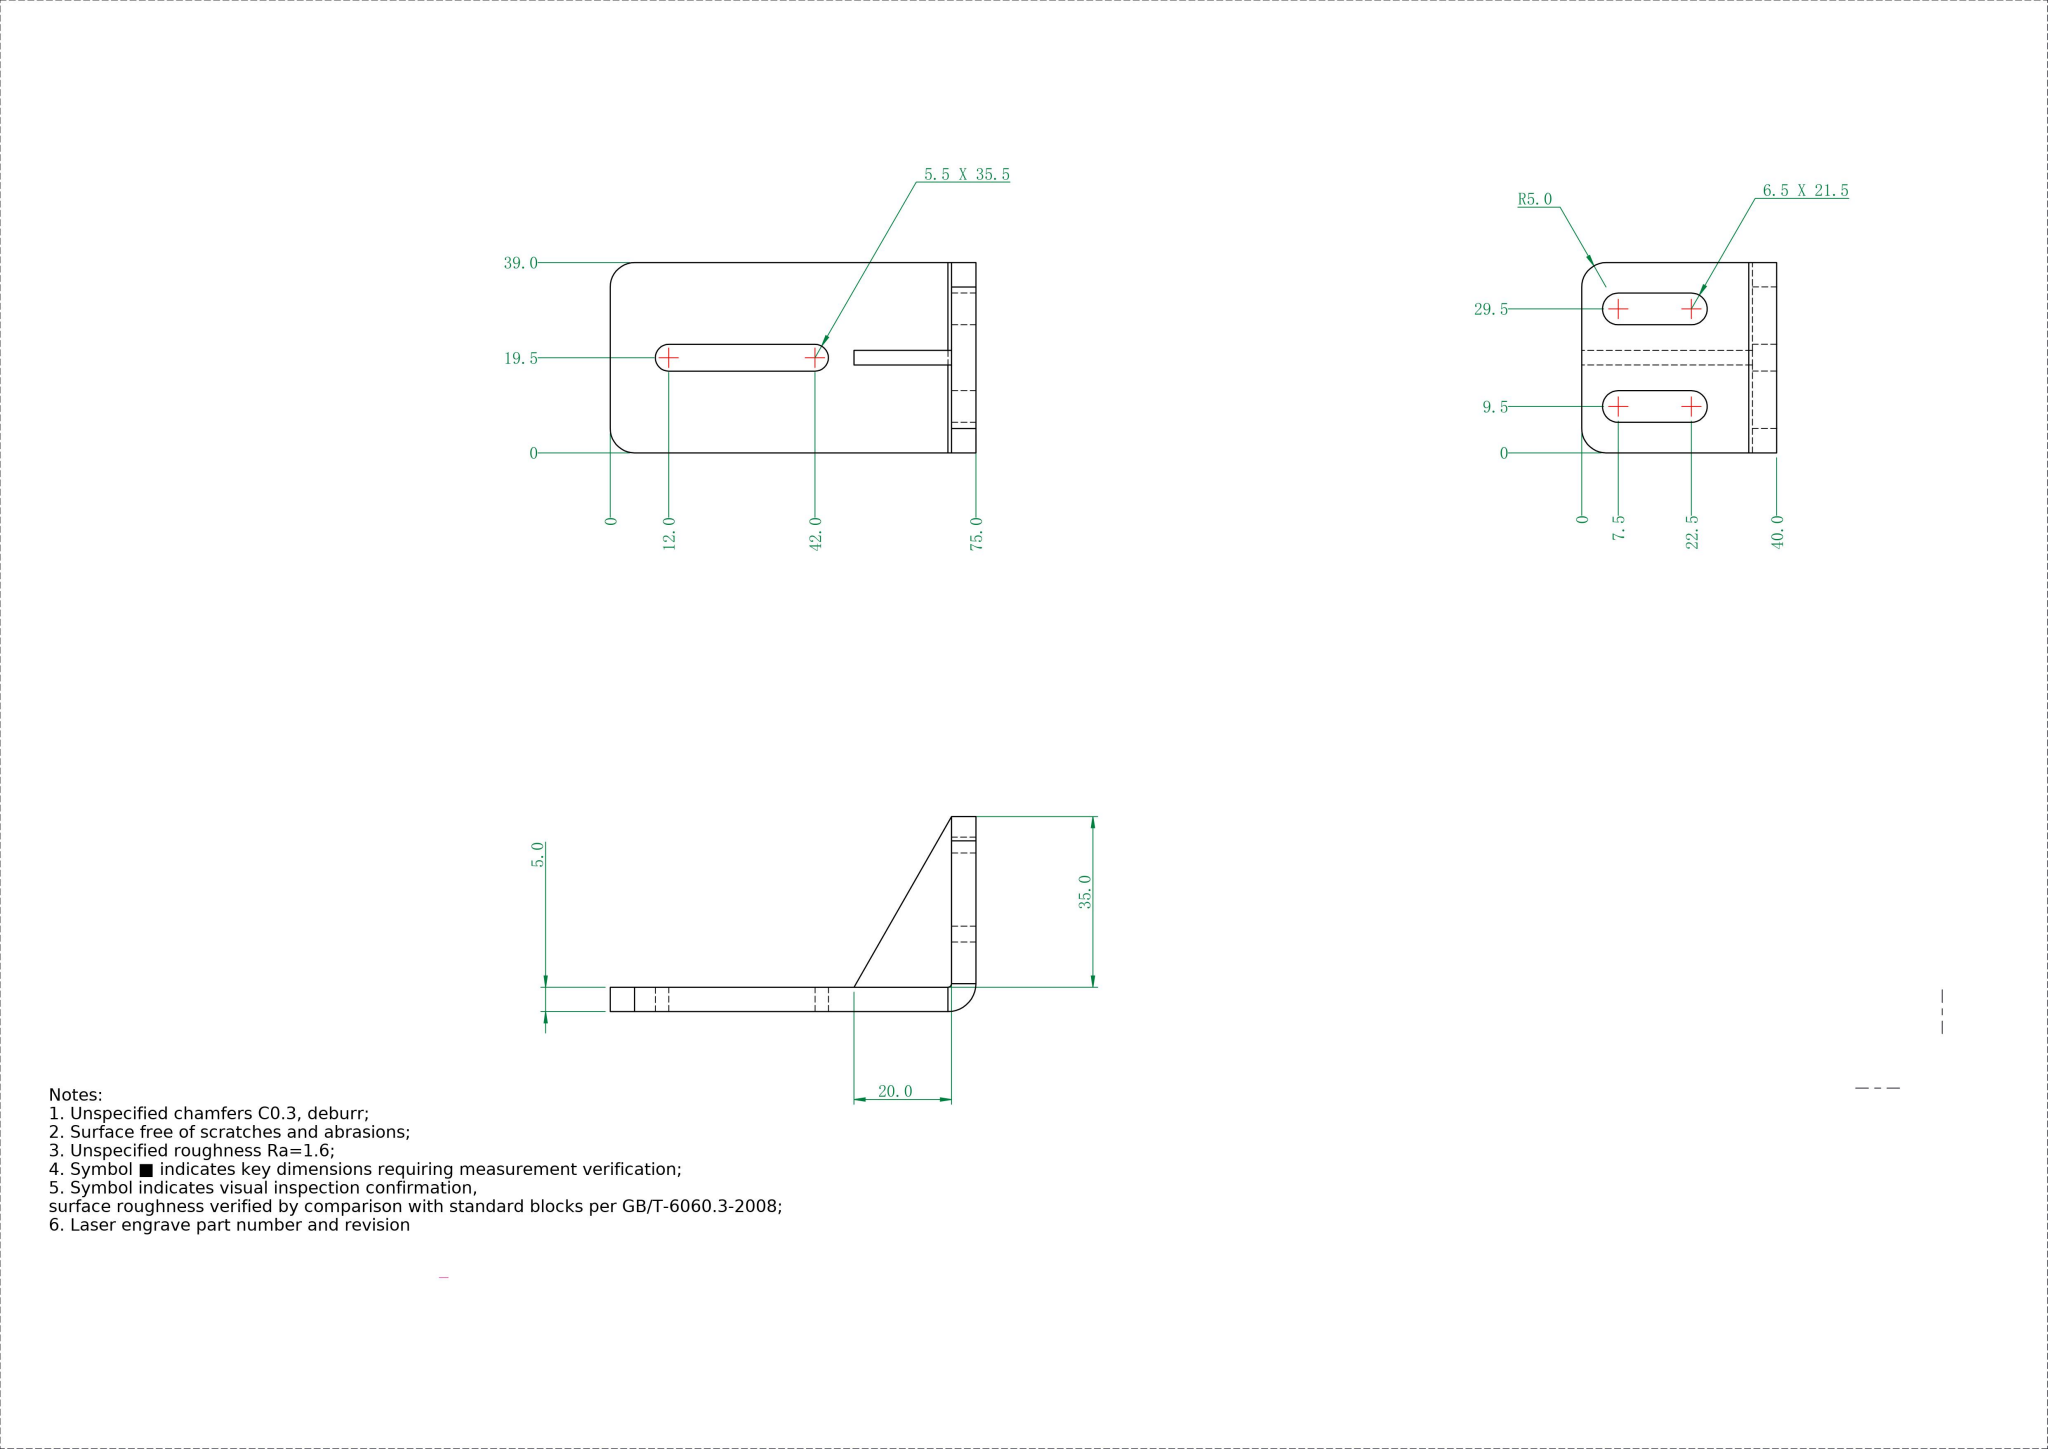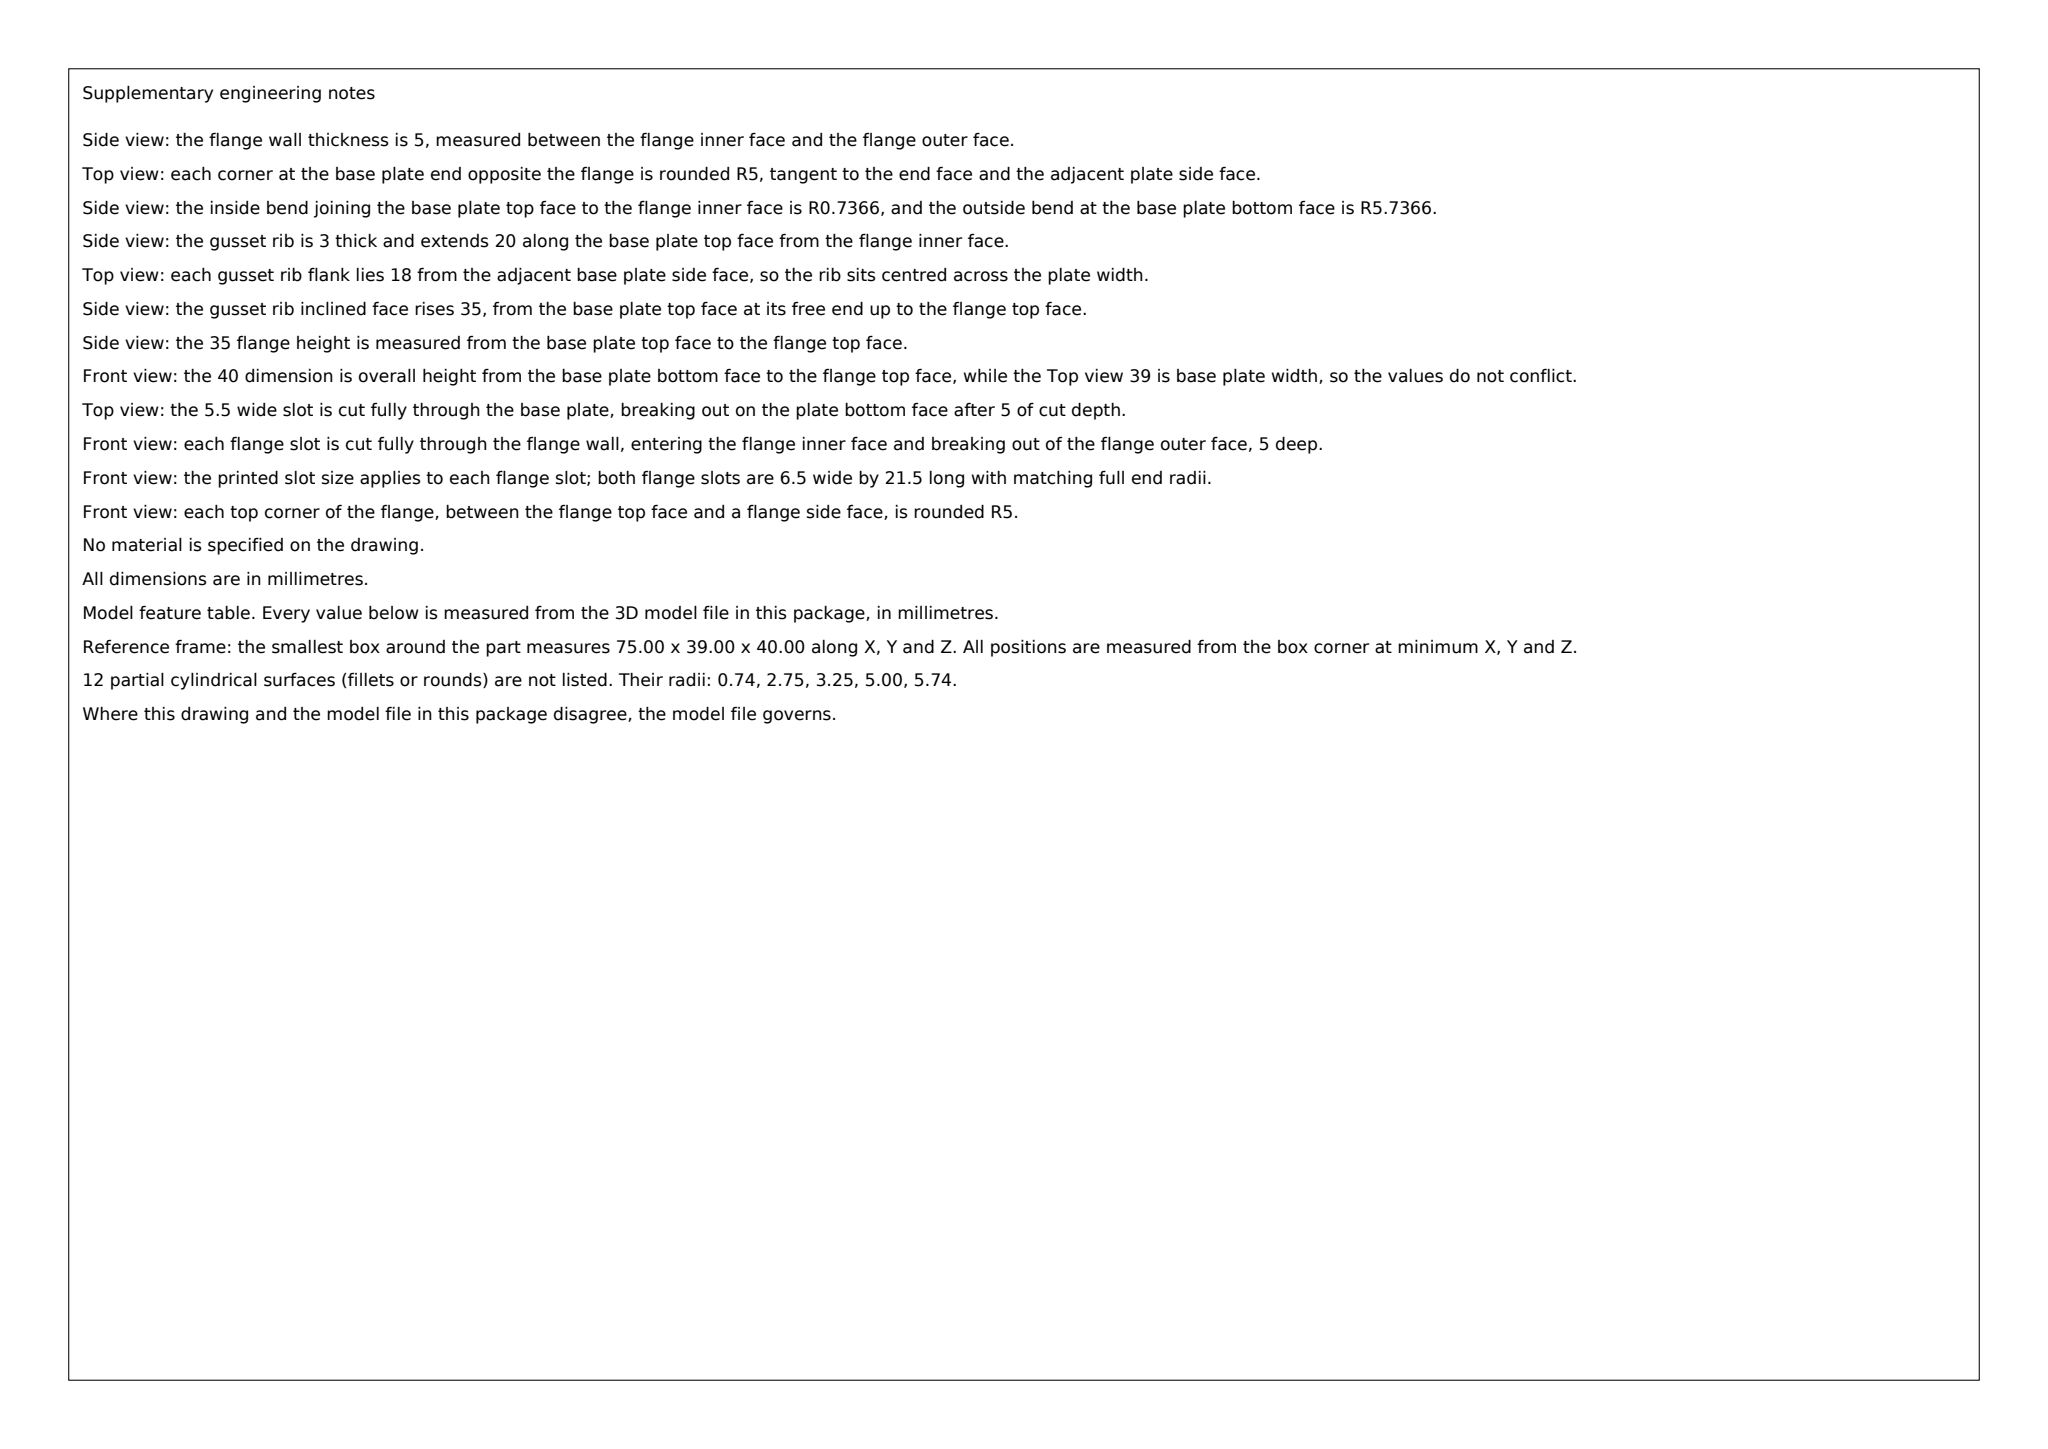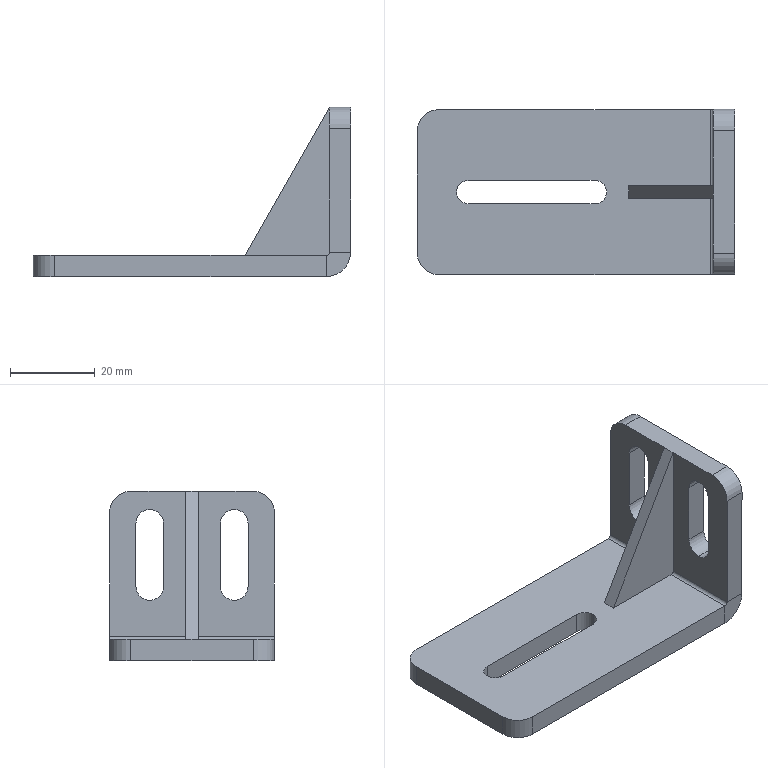Part | SolidWorks | mm | 1 solid | 38 faces | box 75 x 39 x 40 mm | volume 19871 mm3 | plane 22 | cylinder 16 | commonest cylinder face diameters 6.5 x6 10 x4 5.5 x3 1.473 x2 11.473 x1
Drawing notes:
GUSSET RIB 3.0 THK SYM ABOUT 39 WIDTH CL (Y 18.0-21.0) | from the solid: Rib faces y=18.0 & 21.0, x 50-70, z 5-40; part width y 0-39, CL=19.5
UPRIGHT LEG HT 35.0 ABOVE BASE TOP FACE; 40.0 OVERALL | from the solid: Top face z=40.0; base top face z=5.0 (plane z=5, x0-69.3, y0-39); bbox Z=40.0